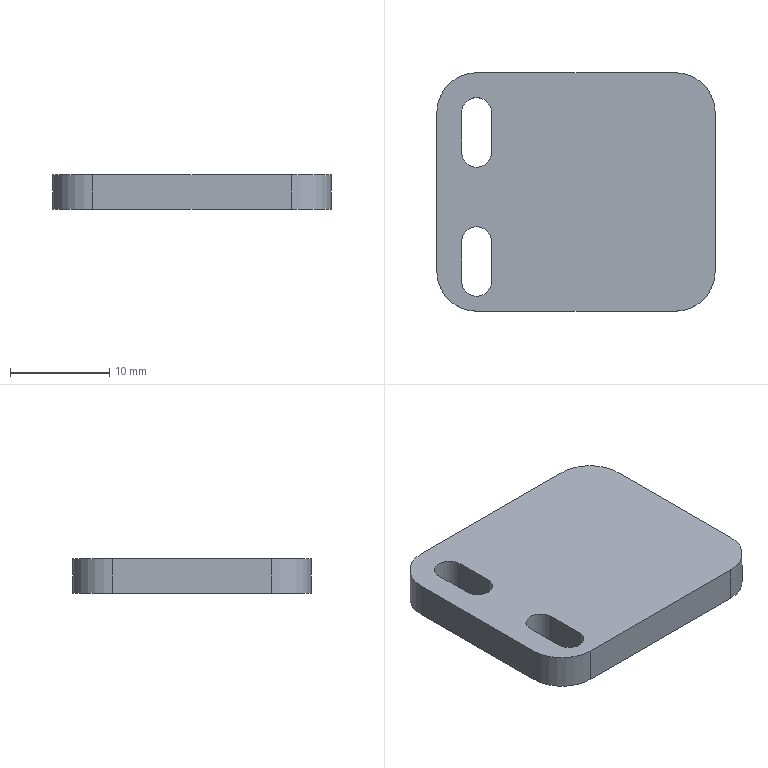CAM job | Mastercam | mm | 7 operations | part box 28 x 24 x 3.5
1. Contour (Ramp) | 6 - 6 平底刀
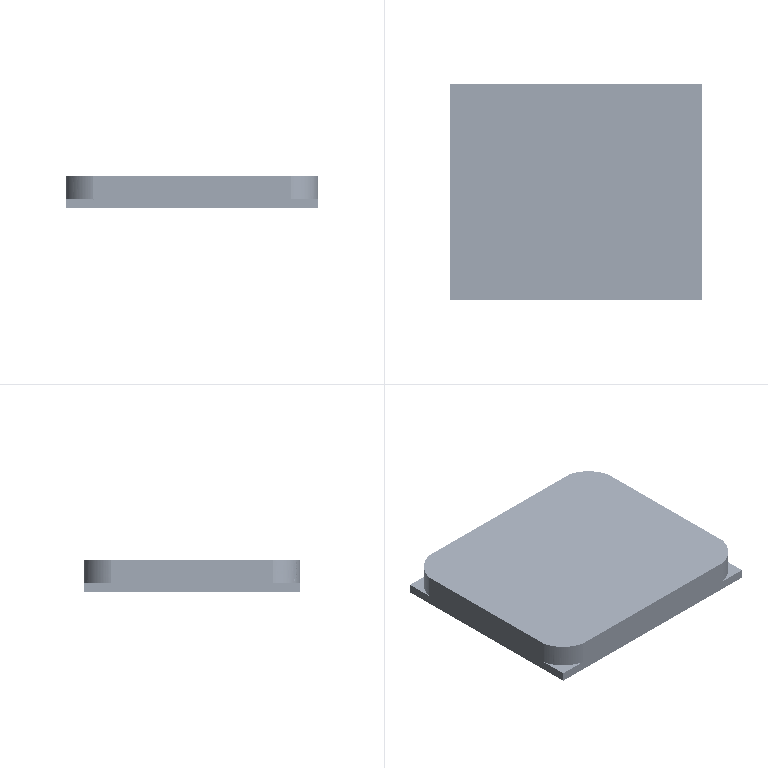2. Facing | 7 - 4 平底刀
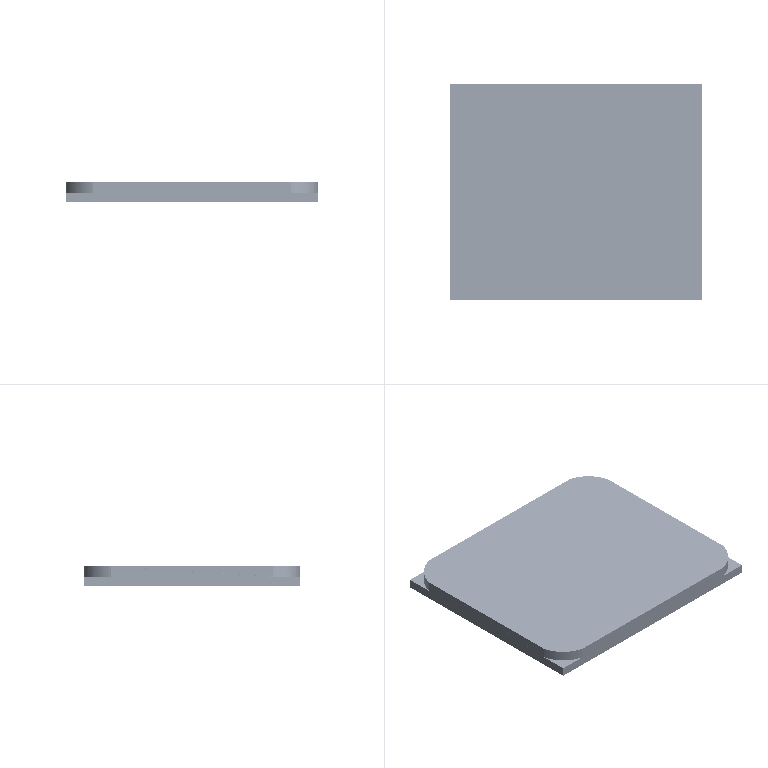3. Facing | 7 - 4 平底刀
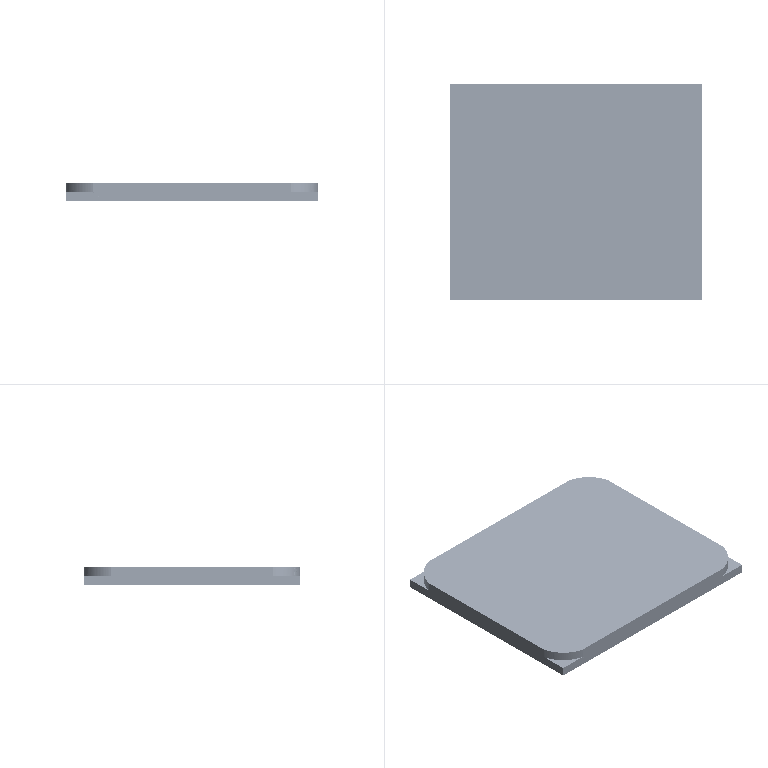4. Contour (Ramp) | 17 - 2 平铣刀
5. Contour (Ramp) | 6 - 6 平底刀
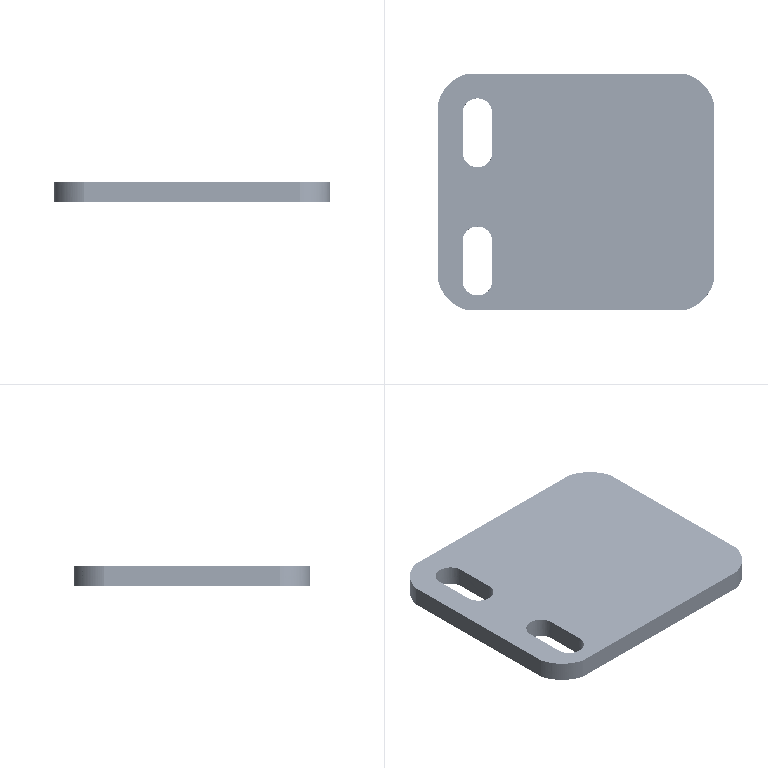6. Contour (2D) | 7 - 4 平底刀
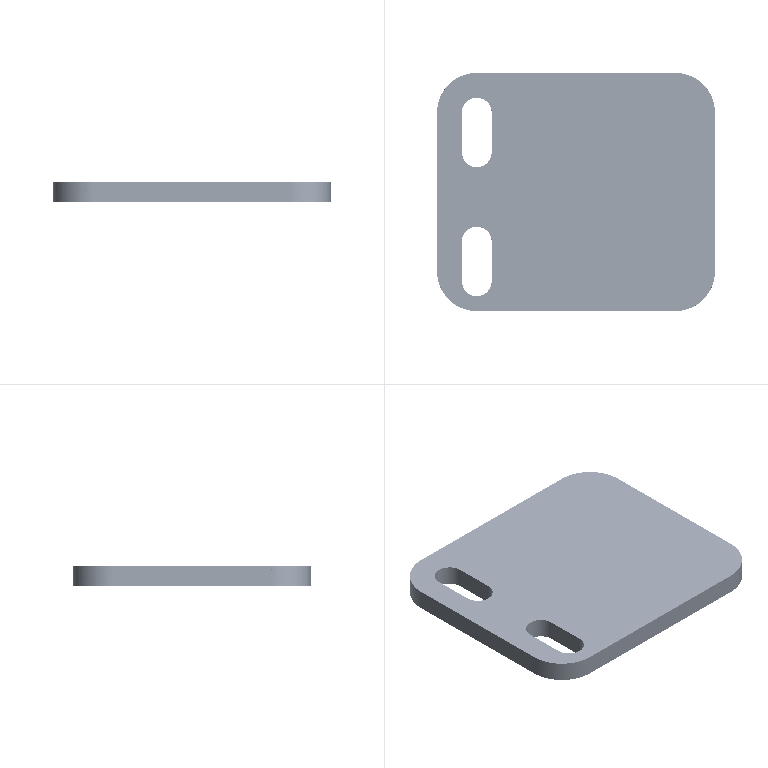7. Model Chamfer | 2 - 6定位倒角